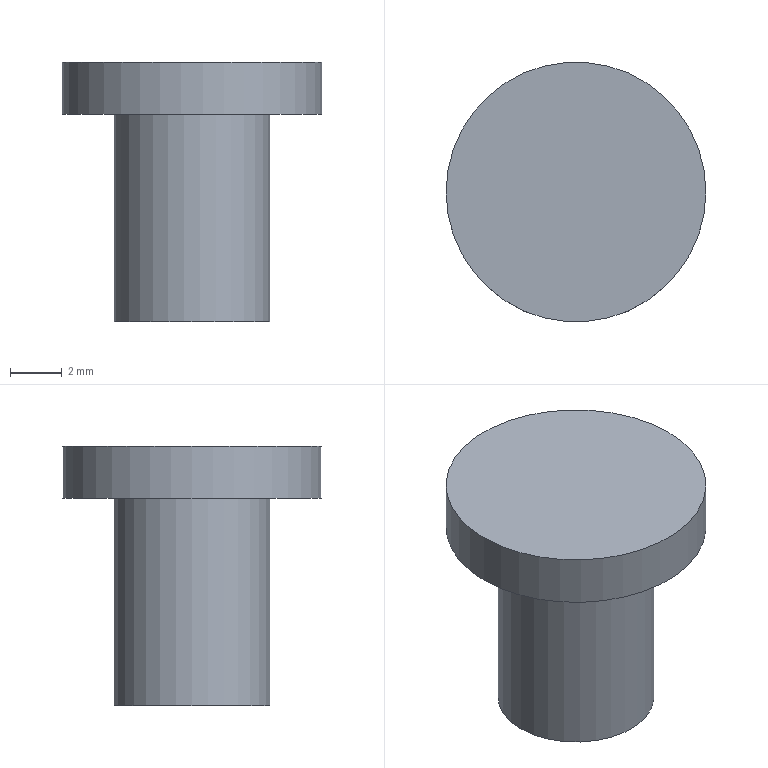Component | NX | 1 | 1 solid | 5 faces | box 10 x 10 x 10 mm | volume 383 mm3 | plane 3 | cylinder 2 | commonest cylinder face diameters 10 x1 6 x1
STEP:
#1=CARTESIAN_POINT('',(0.,0.,0.));
#2=DIRECTION('',(0.,0.,1.));
#3=DIRECTION('',(1.,0.,0.));
#4=AXIS2_PLACEMENT_3D('',#1,#2,#3);
#5=CARTESIAN_POINT('',(43.,-25.,6.));
#6=VERTEX_POINT('',#5);
#7=CARTESIAN_POINT('',(40.,-25.,6.));
#8=DIRECTION('',(0.,0.,-1.));
#9=DIRECTION('',(1.,0.,0.));
#10=AXIS2_PLACEMENT_3D('',#7,#8,#9);
#11=CIRCLE('',#10,3.);
#12=CARTESIAN_POINT('',(40.,-25.,6.));
#13=DIRECTION('',(0.,0.,-1.));
#14=DIRECTION('',(1.,0.,0.));
#15=AXIS2_PLACEMENT_3D('',#12,#13,#14);
#16=PLANE('',#15);
#17=CARTESIAN_POINT('',(0.,0.));
#18=DIRECTION('',(1.,0.));
#19=AXIS2_PLACEMENT_2D('',#17,#18);
#20=CIRCLE('',#19,3.);
#21=(GEOMETRIC_REPRESENTATION_CONTEXT(2)PARAMETRIC_REPRESENTATION_CONTEXT()REPRESENTATION_CONTEXT('',''));
#22=DEFINITIONAL_REPRESENTATION('',(#20),#21);
#23=PCURVE('',#16,#22);
#24=CARTESIAN_POINT('',(40.,-25.,6.));
#25=DIRECTION('',(0.,0.,-1.));
#26=DIRECTION('',(1.,0.,0.));
#27=AXIS2_PLACEMENT_3D('',#24,#25,#26);
#28=CYLINDRICAL_SURFACE('',#27,3.);
#29=CARTESIAN_POINT('',(0.,0.));
#30=DIRECTION('',(1.,0.));
#31=VECTOR('',#30,1.);
#32=LINE('',#29,#31);
#33=(GEOMETRIC_REPRESENTATION_CONTEXT(2)PARAMETRIC_REPRESENTATION_CONTEXT()REPRESENTATION_CONTEXT('',''));
#34=DEFINITIONAL_REPRESENTATION('',(#32),#33);
#35=PCURVE('',#28,#34);
#36=SURFACE_CURVE('',#11,(#23,#35),.PCURVE_S1.);
#37=EDGE_CURVE('',#6,#6,#36,.T.);
#38=ORIENTED_EDGE('',*,*,#37,.F.);
#39=EDGE_LOOP('',(#38));
#40=FACE_BOUND('',#39,.T.);
#41=CARTESIAN_POINT('',(45.,-25.,6.));
#42=VERTEX_POINT('',#41);
#43=CARTESIAN_POINT('',(40.,-25.,6.));
#44=DIRECTION('',(0.,0.,1.));
#45=DIRECTION('',(1.,0.,0.));
#46=AXIS2_PLACEMENT_3D('',#43,#44,#45);
#47=CIRCLE('',#46,5.);
#48=CARTESIAN_POINT('',(5.,0.));
#49=CARTESIAN_POINT('',(5.,-8.66));
#50=CARTESIAN_POINT('',(-2.5,-4.33));
#51=CARTESIAN_POINT('',(-10.,-0.));
#52=CARTESIAN_POINT('',(-2.5,4.33));
#53=CARTESIAN_POINT('',(5.,8.66));
#54=CARTESIAN_POINT('',(5.,0.));
#55=(BOUNDED_CURVE()B_SPLINE_CURVE(2,(#48,#49,#50,#51,#52,#53,#54),.UNSPECIFIED.,.T.,.F.)B_SPLINE_CURVE_WITH_KNOTS((1,2,2,2,2,1),(-2.094,0.,2.094,4.189,6.283,8.378),.UNSPECIFIED.)CURVE()GEOMETRIC_REPRESENTATION_ITEM()RATIONAL_B_SPLINE_CURVE((1.,0.5,1.,0.5,1.,0.5,1.))REPRESENTATION_ITEM(''));
#56=(GEOMETRIC_REPRESENTATION_CONTEXT(2)PARAMETRIC_REPRESENTATION_CONTEXT()REPRESENTATION_CONTEXT('',''));
#57=DEFINITIONAL_REPRESENTATION('',(#55),#56);
#58=PCURVE('',#16,#57);
#59=CARTESIAN_POINT('',(40.,-25.,8.));
#60=DIRECTION('',(0.,0.,-1.));
#61=DIRECTION('',(1.,0.,0.));
#62=AXIS2_PLACEMENT_3D('',#59,#60,#61);
#63=CYLINDRICAL_SURFACE('',#62,5.);
#64=CARTESIAN_POINT('',(6.283,2.));
#65=DIRECTION('',(-1.,0.));
#66=VECTOR('',#65,1.);
#67=LINE('',#64,#66);
#68=(GEOMETRIC_REPRESENTATION_CONTEXT(2)PARAMETRIC_REPRESENTATION_CONTEXT()REPRESENTATION_CONTEXT('',''));
#69=DEFINITIONAL_REPRESENTATION('',(#67),#68);
#70=PCURVE('',#63,#69);
#71=SURFACE_CURVE('',#47,(#58,#70),.PCURVE_S1.);
#72=EDGE_CURVE('',#42,#42,#71,.T.);
#73=ORIENTED_EDGE('',*,*,#72,.F.);
#74=EDGE_LOOP('',(#73));
#75=FACE_BOUND('',#74,.T.);
#76=ADVANCED_FACE('',(#40,#75),#16,.T.);
#77=CARTESIAN_POINT('',(45.,-25.,8.));
#78=VERTEX_POINT('',#77);
#79=CARTESIAN_POINT('',(40.,-25.,8.));
#80=DIRECTION('',(0.,0.,-1.));
#81=DIRECTION('',(1.,0.,0.));
#82=AXIS2_PLACEMENT_3D('',#79,#80,#81);
#83=CIRCLE('',#82,5.);
#84=CARTESIAN_POINT('',(40.,-25.,8.));
#85=DIRECTION('',(0.,0.,1.));
#86=DIRECTION('',(-1.,0.,0.));
#87=AXIS2_PLACEMENT_3D('',#84,#85,#86);
#88=PLANE('',#87);
#89=CARTESIAN_POINT('',(-5.,0.));
#90=CARTESIAN_POINT('',(-5.,8.66));
#91=CARTESIAN_POINT('',(2.5,4.33));
#92=CARTESIAN_POINT('',(10.,0.));
#93=CARTESIAN_POINT('',(2.5,-4.33));
#94=CARTESIAN_POINT('',(-5.,-8.66));
#95=CARTESIAN_POINT('',(-5.,0.));
#96=(BOUNDED_CURVE()B_SPLINE_CURVE(2,(#89,#90,#91,#92,#93,#94,#95),.UNSPECIFIED.,.T.,.F.)B_SPLINE_CURVE_WITH_KNOTS((1,2,2,2,2,1),(-2.094,0.,2.094,4.189,6.283,8.378),.UNSPECIFIED.)CURVE()GEOMETRIC_REPRESENTATION_ITEM()RATIONAL_B_SPLINE_CURVE((1.,0.5,1.,0.5,1.,0.5,1.))REPRESENTATION_ITEM(''));
#97=(GEOMETRIC_REPRESENTATION_CONTEXT(2)PARAMETRIC_REPRESENTATION_CONTEXT()REPRESENTATION_CONTEXT('',''));
#98=DEFINITIONAL_REPRESENTATION('',(#96),#97);
#99=PCURVE('',#88,#98);
#100=CARTESIAN_POINT('',(0.,0.));
#101=DIRECTION('',(1.,0.));
#102=VECTOR('',#101,1.);
#103=LINE('',#100,#102);
#104=(GEOMETRIC_REPRESENTATION_CONTEXT(2)PARAMETRIC_REPRESENTATION_CONTEXT()REPRESENTATION_CONTEXT('',''));
#105=DEFINITIONAL_REPRESENTATION('',(#103),#104);
#106=PCURVE('',#63,#105);
#107=SURFACE_CURVE('',#83,(#99,#106),.PCURVE_S1.);
#108=EDGE_CURVE('',#78,#78,#107,.T.);
#109=ORIENTED_EDGE('',*,*,#108,.F.);
#110=EDGE_LOOP('',(#109));
#111=FACE_BOUND('',#110,.T.);
#112=ADVANCED_FACE('',(#111),#88,.T.);
#113=ORIENTED_EDGE('',*,*,#72,.T.);
#114=CARTESIAN_POINT('',(45.,-25.,8.));
#115=CARTESIAN_POINT('',(45.,-25.,6.));
#116=B_SPLINE_CURVE_WITH_KNOTS('',1,(#114,#115),.UNSPECIFIED.,.F.,.F.,(2,2),(0.,2.),.PIECEWISE_BEZIER_KNOTS.);
#117=CARTESIAN_POINT('',(0.,0.));
#118=DIRECTION('',(0.,1.));
#119=VECTOR('',#118,1.);
#120=LINE('',#117,#119);
#121=(GEOMETRIC_REPRESENTATION_CONTEXT(2)PARAMETRIC_REPRESENTATION_CONTEXT()REPRESENTATION_CONTEXT('',''));
#122=DEFINITIONAL_REPRESENTATION('',(#120),#121);
#123=PCURVE('',#63,#122);
#124=CARTESIAN_POINT('',(6.283,0.));
#125=DIRECTION('',(0.,1.));
#126=VECTOR('',#125,1.);
#127=LINE('',#124,#126);
#128=(GEOMETRIC_REPRESENTATION_CONTEXT(2)PARAMETRIC_REPRESENTATION_CONTEXT()REPRESENTATION_CONTEXT('',''));
#129=DEFINITIONAL_REPRESENTATION('',(#127),#128);
#130=PCURVE('',#63,#129);
#131=SEAM_CURVE('',#116,(#123,#130),.PCURVE_S1.);
#132=EDGE_CURVE('',#78,#42,#131,.T.);
#133=ORIENTED_EDGE('',*,*,#132,.F.);
#134=ORIENTED_EDGE('',*,*,#108,.T.);
#135=ORIENTED_EDGE('',*,*,#132,.T.);
#136=EDGE_LOOP('',(#113,#133,#134,#135));
#137=FACE_BOUND('',#136,.T.);
#138=ADVANCED_FACE('',(#137),#63,.T.);
#139=CARTESIAN_POINT('',(43.,-25.,-2.));
#140=VERTEX_POINT('',#139);
#141=CARTESIAN_POINT('',(40.,-25.,-2.));
#142=DIRECTION('',(0.,0.,1.));
#143=DIRECTION('',(1.,0.,0.));
#144=AXIS2_PLACEMENT_3D('',#141,#142,#143);
#145=CIRCLE('',#144,3.);
#146=CARTESIAN_POINT('',(40.,-25.,-2.));
#147=DIRECTION('',(0.,0.,-1.));
#148=DIRECTION('',(1.,0.,0.));
#149=AXIS2_PLACEMENT_3D('',#146,#147,#148);
#150=PLANE('',#149);
#151=CARTESIAN_POINT('',(3.,0.));
#152=CARTESIAN_POINT('',(3.,-5.196));
#153=CARTESIAN_POINT('',(-1.5,-2.598));
#154=CARTESIAN_POINT('',(-6.,-0.));
#155=CARTESIAN_POINT('',(-1.5,2.598));
#156=CARTESIAN_POINT('',(3.,5.196));
#157=CARTESIAN_POINT('',(3.,0.));
#158=(BOUNDED_CURVE()B_SPLINE_CURVE(2,(#151,#152,#153,#154,#155,#156,#157),.UNSPECIFIED.,.T.,.F.)B_SPLINE_CURVE_WITH_KNOTS((1,2,2,2,2,1),(-2.094,0.,2.094,4.189,6.283,8.378),.UNSPECIFIED.)CURVE()GEOMETRIC_REPRESENTATION_ITEM()RATIONAL_B_SPLINE_CURVE((1.,0.5,1.,0.5,1.,0.5,1.))REPRESENTATION_ITEM(''));
#159=(GEOMETRIC_REPRESENTATION_CONTEXT(2)PARAMETRIC_REPRESENTATION_CONTEXT()REPRESENTATION_CONTEXT('',''));
#160=DEFINITIONAL_REPRESENTATION('',(#158),#159);
#161=PCURVE('',#150,#160);
#162=CARTESIAN_POINT('',(6.283,8.));
#163=DIRECTION('',(-1.,0.));
#164=VECTOR('',#163,1.);
#165=LINE('',#162,#164);
#166=(GEOMETRIC_REPRESENTATION_CONTEXT(2)PARAMETRIC_REPRESENTATION_CONTEXT()REPRESENTATION_CONTEXT('',''));
#167=DEFINITIONAL_REPRESENTATION('',(#165),#166);
#168=PCURVE('',#28,#167);
#169=SURFACE_CURVE('',#145,(#161,#168),.PCURVE_S1.);
#170=EDGE_CURVE('',#140,#140,#169,.T.);
#171=ORIENTED_EDGE('',*,*,#170,.F.);
#172=EDGE_LOOP('',(#171));
#173=FACE_BOUND('',#172,.T.);
#174=ADVANCED_FACE('',(#173),#150,.T.);
#175=ORIENTED_EDGE('',*,*,#170,.T.);
#176=CARTESIAN_POINT('',(43.,-25.,6.));
#177=CARTESIAN_POINT('',(43.,-25.,-2.));
#178=B_SPLINE_CURVE_WITH_KNOTS('',1,(#176,#177),.UNSPECIFIED.,.F.,.F.,(2,2),(0.,8.),.PIECEWISE_BEZIER_KNOTS.);
#179=CARTESIAN_POINT('',(0.,0.));
#180=DIRECTION('',(0.,1.));
#181=VECTOR('',#180,1.);
#182=LINE('',#179,#181);
#183=(GEOMETRIC_REPRESENTATION_CONTEXT(2)PARAMETRIC_REPRESENTATION_CONTEXT()REPRESENTATION_CONTEXT('',''));
#184=DEFINITIONAL_REPRESENTATION('',(#182),#183);
#185=PCURVE('',#28,#184);
#186=CARTESIAN_POINT('',(6.283,0.));
#187=DIRECTION('',(0.,1.));
#188=VECTOR('',#187,1.);
#189=LINE('',#186,#188);
#190=(GEOMETRIC_REPRESENTATION_CONTEXT(2)PARAMETRIC_REPRESENTATION_CONTEXT()REPRESENTATION_CONTEXT('',''));
#191=DEFINITIONAL_REPRESENTATION('',(#189),#190);
#192=PCURVE('',#28,#191);
#193=SEAM_CURVE('',#178,(#185,#192),.PCURVE_S1.);
#194=EDGE_CURVE('',#6,#140,#193,.T.);
#195=ORIENTED_EDGE('',*,*,#194,.F.);
#196=ORIENTED_EDGE('',*,*,#37,.T.);
#197=ORIENTED_EDGE('',*,*,#194,.T.);
#198=EDGE_LOOP('',(#175,#195,#196,#197));
#199=FACE_BOUND('',#198,.T.);
#200=ADVANCED_FACE('',(#199),#28,.T.);
#201=CLOSED_SHELL('',(#76,#112,#138,#174,#200));
#202=MANIFOLD_SOLID_BREP('',#201);
#203=(LENGTH_UNIT()NAMED_UNIT(*)SI_UNIT(.MILLI.,.METRE.));
#204=UNCERTAINTY_MEASURE_WITH_UNIT(LENGTH_MEASURE(0.00001),#203,'','');
#205=(NAMED_UNIT(*)PLANE_ANGLE_UNIT()SI_UNIT($,.RADIAN.));
#206=(NAMED_UNIT(*)SI_UNIT($,.STERADIAN.)SOLID_ANGLE_UNIT());
#207=(GEOMETRIC_REPRESENTATION_CONTEXT(3)GLOBAL_UNCERTAINTY_ASSIGNED_CONTEXT((#204))GLOBAL_UNIT_ASSIGNED_CONTEXT((#203,#205,#206))REPRESENTATION_CONTEXT('',''));
#208=ADVANCED_BREP_SHAPE_REPRESENTATION('',(#4,#202),#207);